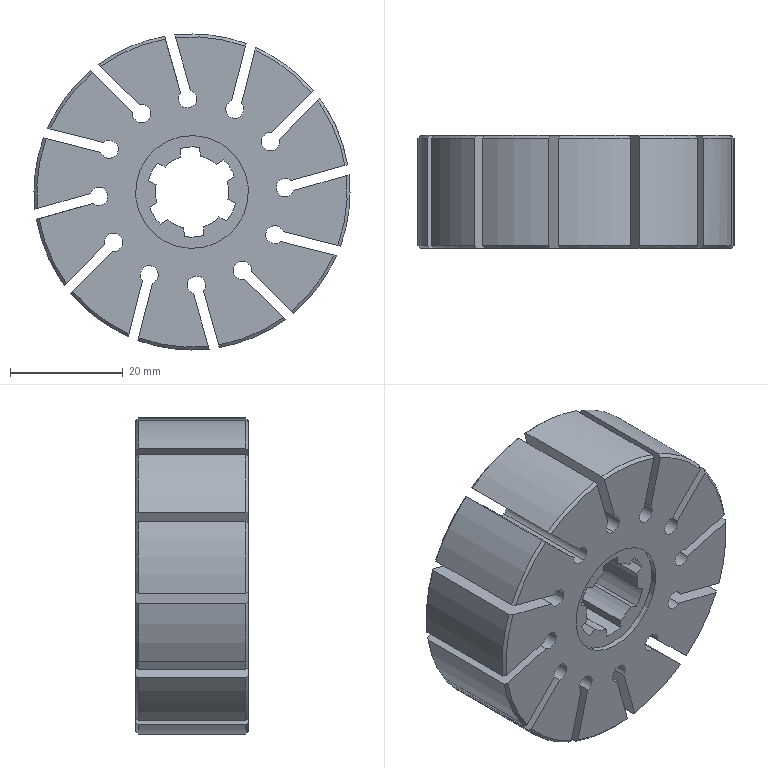Component | SolidWorks | 4-1 | 1 solid | 120 faces | volume 39312 mm3 | cylinder 54 | plane 40 | cone 26 | commonest cylinder face diameters 3.2 x24 56 x13 16 x7 13 x6 20 x4